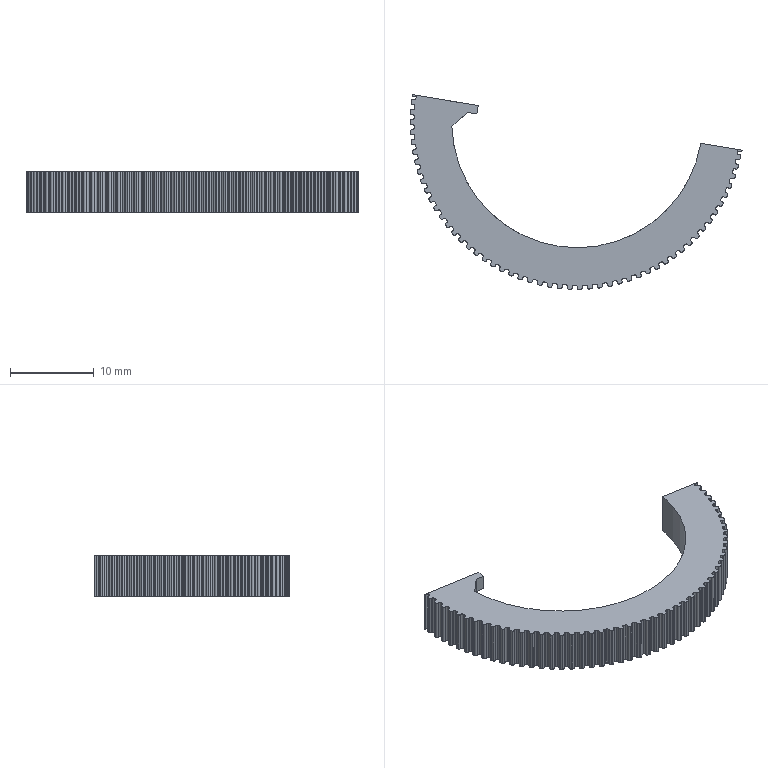Component | NX | INTERNAL_STRUCTURE | 1 solid | 424 faces | volume 1298 mm3 | cylinder 310 | plane 114 | commonest cylinder face diameters 0.4 x204 40 x53 39 x52 30 x1